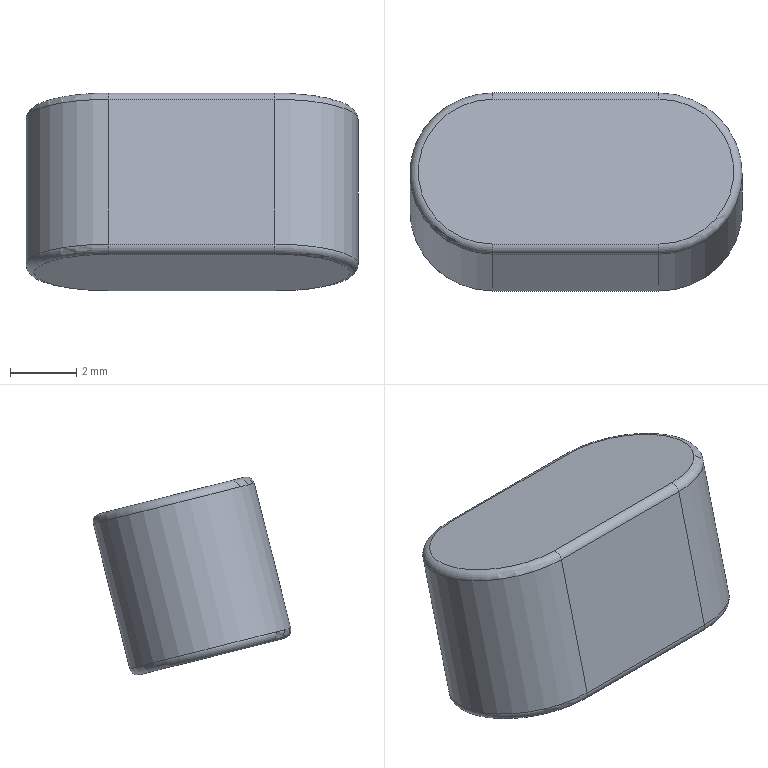Component | NX | STANDARD_FLAT_KEY_A_5X5X10 | 1 solid | 14 faces | box 10 x 5.96 x 5.96 mm | volume 222 mm3 | cylinder 6 | plane 4 | torus 4 | commonest cylinder face diameters 0.5 x4 5 x2
STEP:
#1=CARTESIAN_POINT('',(0.,0.,0.));
#2=DIRECTION('',(0.,0.,1.));
#3=DIRECTION('',(1.,0.,0.));
#4=AXIS2_PLACEMENT_3D('',#1,#2,#3);
#5=CARTESIAN_POINT('',(-1.948,67.926,64.209));
#6=VERTEX_POINT('',#5);
#7=CARTESIAN_POINT('',(-1.948,69.023,68.574));
#8=VERTEX_POINT('',#7);
#9=CARTESIAN_POINT('',(-1.948,67.865,63.967));
#10=DIRECTION('',(0.,0.2438,0.9698));
#11=VECTOR('',#10,1.);
#12=LINE('',#9,#11);
#13=CARTESIAN_POINT('',(-1.948,67.865,63.967));
#14=DIRECTION('',(0.,0.9698,-0.2438));
#15=DIRECTION('',(1.,-0.,0.));
#16=AXIS2_PLACEMENT_3D('',#13,#14,#15);
#17=PLANE('',#16);
#18=CARTESIAN_POINT('',(0.,0.));
#19=DIRECTION('',(-0.,-1.));
#20=VECTOR('',#19,1.);
#21=LINE('',#18,#20);
#22=(GEOMETRIC_REPRESENTATION_CONTEXT(2)PARAMETRIC_REPRESENTATION_CONTEXT()REPRESENTATION_CONTEXT('',''));
#23=DEFINITIONAL_REPRESENTATION('',(#21),#22);
#24=PCURVE('',#17,#23);
#25=CARTESIAN_POINT('',(-1.948,65.44,64.576));
#26=DIRECTION('',(0.,0.2438,0.9698));
#27=DIRECTION('',(-1.,0.,0.));
#28=AXIS2_PLACEMENT_3D('',#25,#26,#27);
#29=CYLINDRICAL_SURFACE('',#28,2.5);
#30=CARTESIAN_POINT('',(4.712,-0.));
#31=DIRECTION('',(0.,1.));
#32=VECTOR('',#31,1.);
#33=LINE('',#30,#32);
#34=(GEOMETRIC_REPRESENTATION_CONTEXT(2)PARAMETRIC_REPRESENTATION_CONTEXT()REPRESENTATION_CONTEXT('',''));
#35=DEFINITIONAL_REPRESENTATION('',(#33),#34);
#36=PCURVE('',#29,#35);
#37=SURFACE_CURVE('',#12,(#24,#36),.PCURVE_S1.);
#38=EDGE_CURVE('',#6,#8,#37,.T.);
#39=ORIENTED_EDGE('',*,*,#38,.F.);
#40=CARTESIAN_POINT('',(-6.948,67.926,64.209));
#41=VERTEX_POINT('',#40);
#42=CARTESIAN_POINT('',(-6.948,67.926,64.209));
#43=DIRECTION('',(-1.,0.,-0.));
#44=VECTOR('',#43,1.);
#45=LINE('',#42,#44);
#46=CARTESIAN_POINT('',(-5.,-0.25));
#47=DIRECTION('',(-1.,0.));
#48=VECTOR('',#47,1.);
#49=LINE('',#46,#48);
#50=(GEOMETRIC_REPRESENTATION_CONTEXT(2)PARAMETRIC_REPRESENTATION_CONTEXT()REPRESENTATION_CONTEXT('',''));
#51=DEFINITIONAL_REPRESENTATION('',(#49),#50);
#52=PCURVE('',#17,#51);
#53=CARTESIAN_POINT('',(-1.948,67.683,64.27));
#54=DIRECTION('',(1.,-0.,0.));
#55=DIRECTION('',(-0.,-0.9698,0.2438));
#56=AXIS2_PLACEMENT_3D('',#53,#54,#55);
#57=CYLINDRICAL_SURFACE('',#56,0.25);
#58=CARTESIAN_POINT('',(3.142,-5.));
#59=DIRECTION('',(0.,-1.));
#60=VECTOR('',#59,1.);
#61=LINE('',#58,#60);
#62=(GEOMETRIC_REPRESENTATION_CONTEXT(2)PARAMETRIC_REPRESENTATION_CONTEXT()REPRESENTATION_CONTEXT('',''));
#63=DEFINITIONAL_REPRESENTATION('',(#61),#62);
#64=PCURVE('',#57,#63);
#65=SURFACE_CURVE('',#45,(#52,#64),.PCURVE_S1.);
#66=EDGE_CURVE('',#6,#41,#65,.T.);
#67=ORIENTED_EDGE('',*,*,#66,.T.);
#68=CARTESIAN_POINT('',(-6.948,69.023,68.574));
#69=VERTEX_POINT('',#68);
#70=CARTESIAN_POINT('',(-6.948,67.865,63.967));
#71=DIRECTION('',(0.,0.2438,0.9698));
#72=VECTOR('',#71,1.);
#73=LINE('',#70,#72);
#74=CARTESIAN_POINT('',(-5.,0.));
#75=DIRECTION('',(-0.,-1.));
#76=VECTOR('',#75,1.);
#77=LINE('',#74,#76);
#78=(GEOMETRIC_REPRESENTATION_CONTEXT(2)PARAMETRIC_REPRESENTATION_CONTEXT()REPRESENTATION_CONTEXT('',''));
#79=DEFINITIONAL_REPRESENTATION('',(#77),#78);
#80=PCURVE('',#17,#79);
#81=CARTESIAN_POINT('',(-6.948,65.44,64.576));
#82=DIRECTION('',(0.,0.2438,0.9698));
#83=DIRECTION('',(-1.,0.,0.));
#84=AXIS2_PLACEMENT_3D('',#81,#82,#83);
#85=CYLINDRICAL_SURFACE('',#84,2.5);
#86=CARTESIAN_POINT('',(-1.571,-0.));
#87=DIRECTION('',(0.,1.));
#88=VECTOR('',#87,1.);
#89=LINE('',#86,#88);
#90=(GEOMETRIC_REPRESENTATION_CONTEXT(2)PARAMETRIC_REPRESENTATION_CONTEXT()REPRESENTATION_CONTEXT('',''));
#91=DEFINITIONAL_REPRESENTATION('',(#89),#90);
#92=PCURVE('',#85,#91);
#93=SURFACE_CURVE('',#73,(#80,#92),.PCURVE_S1.);
#94=EDGE_CURVE('',#41,#69,#93,.T.);
#95=ORIENTED_EDGE('',*,*,#94,.T.);
#96=CARTESIAN_POINT('',(-1.948,69.023,68.574));
#97=DIRECTION('',(1.,-0.,0.));
#98=VECTOR('',#97,1.);
#99=LINE('',#96,#98);
#100=CARTESIAN_POINT('',(-0.,-4.75));
#101=DIRECTION('',(1.,-0.));
#102=VECTOR('',#101,1.);
#103=LINE('',#100,#102);
#104=(GEOMETRIC_REPRESENTATION_CONTEXT(2)PARAMETRIC_REPRESENTATION_CONTEXT()REPRESENTATION_CONTEXT('',''));
#105=DEFINITIONAL_REPRESENTATION('',(#103),#104);
#106=PCURVE('',#17,#105);
#107=CARTESIAN_POINT('',(-6.948,68.78,68.635));
#108=DIRECTION('',(-1.,0.,-0.));
#109=DIRECTION('',(0.,0.9698,-0.2438));
#110=AXIS2_PLACEMENT_3D('',#107,#108,#109);
#111=CYLINDRICAL_SURFACE('',#110,0.25);
#112=CARTESIAN_POINT('',(6.283,-5.));
#113=DIRECTION('',(0.,-1.));
#114=VECTOR('',#113,1.);
#115=LINE('',#112,#114);
#116=(GEOMETRIC_REPRESENTATION_CONTEXT(2)PARAMETRIC_REPRESENTATION_CONTEXT()REPRESENTATION_CONTEXT('',''));
#117=DEFINITIONAL_REPRESENTATION('',(#115),#116);
#118=PCURVE('',#111,#117);
#119=SURFACE_CURVE('',#99,(#106,#118),.PCURVE_S1.);
#120=EDGE_CURVE('',#69,#8,#119,.T.);
#121=ORIENTED_EDGE('',*,*,#120,.T.);
#122=EDGE_LOOP('',(#39,#67,#95,#121));
#123=FACE_BOUND('',#122,.T.);
#124=ADVANCED_FACE('',(#123),#17,.T.);
#125=ORIENTED_EDGE('',*,*,#94,.F.);
#126=CARTESIAN_POINT('',(-6.948,63.077,65.428));
#127=VERTEX_POINT('',#126);
#128=CARTESIAN_POINT('',(-6.948,65.501,64.819));
#129=DIRECTION('',(0.,0.2438,0.9698));
#130=DIRECTION('',(-1.,0.,0.));
#131=AXIS2_PLACEMENT_3D('',#128,#129,#130);
#132=CIRCLE('',#131,2.5);
#133=CARTESIAN_POINT('',(-6.283,0.25));
#134=DIRECTION('',(1.,0.));
#135=VECTOR('',#134,1.);
#136=LINE('',#133,#135);
#137=(GEOMETRIC_REPRESENTATION_CONTEXT(2)PARAMETRIC_REPRESENTATION_CONTEXT()REPRESENTATION_CONTEXT('',''));
#138=DEFINITIONAL_REPRESENTATION('',(#136),#137);
#139=PCURVE('',#85,#138);
#140=CARTESIAN_POINT('',(-6.948,65.501,64.819));
#141=DIRECTION('',(0.,0.2438,0.9698));
#142=DIRECTION('',(-1.,0.,0.));
#143=AXIS2_PLACEMENT_3D('',#140,#141,#142);
#144=TOROIDAL_SURFACE('',#143,2.25,0.25);
#145=CARTESIAN_POINT('',(-6.283,6.283));
#146=DIRECTION('',(1.,0.));
#147=VECTOR('',#146,1.);
#148=LINE('',#145,#147);
#149=(GEOMETRIC_REPRESENTATION_CONTEXT(2)PARAMETRIC_REPRESENTATION_CONTEXT()REPRESENTATION_CONTEXT('',''));
#150=DEFINITIONAL_REPRESENTATION('',(#148),#149);
#151=PCURVE('',#144,#150);
#152=SURFACE_CURVE('',#132,(#139,#151),.PCURVE_S1.);
#153=EDGE_CURVE('',#41,#127,#152,.T.);
#154=ORIENTED_EDGE('',*,*,#153,.T.);
#155=CARTESIAN_POINT('',(-6.948,64.174,69.793));
#156=VERTEX_POINT('',#155);
#157=CARTESIAN_POINT('',(-6.948,63.016,65.186));
#158=DIRECTION('',(0.,0.2438,0.9698));
#159=VECTOR('',#158,1.);
#160=LINE('',#157,#159);
#161=CARTESIAN_POINT('',(1.571,0.));
#162=DIRECTION('',(0.,1.));
#163=VECTOR('',#162,1.);
#164=LINE('',#161,#163);
#165=(GEOMETRIC_REPRESENTATION_CONTEXT(2)PARAMETRIC_REPRESENTATION_CONTEXT()REPRESENTATION_CONTEXT('',''));
#166=DEFINITIONAL_REPRESENTATION('',(#164),#165);
#167=PCURVE('',#85,#166);
#168=CARTESIAN_POINT('',(-6.948,63.016,65.186));
#169=DIRECTION('',(0.,-0.9698,0.2438));
#170=DIRECTION('',(0.,-0.2438,-0.9698));
#171=AXIS2_PLACEMENT_3D('',#168,#169,#170);
#172=PLANE('',#171);
#173=CARTESIAN_POINT('',(-0.,0.));
#174=DIRECTION('',(-1.,0.));
#175=VECTOR('',#174,1.);
#176=LINE('',#173,#175);
#177=(GEOMETRIC_REPRESENTATION_CONTEXT(2)PARAMETRIC_REPRESENTATION_CONTEXT()REPRESENTATION_CONTEXT('',''));
#178=DEFINITIONAL_REPRESENTATION('',(#176),#177);
#179=PCURVE('',#172,#178);
#180=SURFACE_CURVE('',#160,(#167,#179),.PCURVE_S1.);
#181=EDGE_CURVE('',#127,#156,#180,.T.);
#182=ORIENTED_EDGE('',*,*,#181,.T.);
#183=CARTESIAN_POINT('',(-6.948,66.598,69.183));
#184=DIRECTION('',(0.,-0.2438,-0.9698));
#185=DIRECTION('',(-1.,0.,0.));
#186=AXIS2_PLACEMENT_3D('',#183,#184,#185);
#187=CIRCLE('',#186,2.5);
#188=CARTESIAN_POINT('',(6.283,4.75));
#189=DIRECTION('',(-1.,0.));
#190=VECTOR('',#189,1.);
#191=LINE('',#188,#190);
#192=(GEOMETRIC_REPRESENTATION_CONTEXT(2)PARAMETRIC_REPRESENTATION_CONTEXT()REPRESENTATION_CONTEXT('',''));
#193=DEFINITIONAL_REPRESENTATION('',(#191),#192);
#194=PCURVE('',#85,#193);
#195=CARTESIAN_POINT('',(-6.948,66.598,69.183));
#196=DIRECTION('',(0.,0.2438,0.9698));
#197=DIRECTION('',(-1.,0.,0.));
#198=AXIS2_PLACEMENT_3D('',#195,#196,#197);
#199=TOROIDAL_SURFACE('',#198,2.25,0.25);
#200=CARTESIAN_POINT('',(6.283,0.));
#201=DIRECTION('',(-1.,0.));
#202=VECTOR('',#201,1.);
#203=LINE('',#200,#202);
#204=(GEOMETRIC_REPRESENTATION_CONTEXT(2)PARAMETRIC_REPRESENTATION_CONTEXT()REPRESENTATION_CONTEXT('',''));
#205=DEFINITIONAL_REPRESENTATION('',(#203),#204);
#206=PCURVE('',#199,#205);
#207=SURFACE_CURVE('',#187,(#194,#206),.PCURVE_S1.);
#208=EDGE_CURVE('',#156,#69,#207,.T.);
#209=ORIENTED_EDGE('',*,*,#208,.T.);
#210=EDGE_LOOP('',(#125,#154,#182,#209));
#211=FACE_BOUND('',#210,.T.);
#212=ADVANCED_FACE('',(#211),#85,.T.);
#213=ORIENTED_EDGE('',*,*,#181,.F.);
#214=CARTESIAN_POINT('',(-1.948,63.077,65.428));
#215=VERTEX_POINT('',#214);
#216=CARTESIAN_POINT('',(-1.948,63.077,65.428));
#217=DIRECTION('',(1.,0.,0.));
#218=VECTOR('',#217,1.);
#219=LINE('',#216,#218);
#220=CARTESIAN_POINT('',(-0.25,5.));
#221=DIRECTION('',(0.,1.));
#222=VECTOR('',#221,1.);
#223=LINE('',#220,#222);
#224=(GEOMETRIC_REPRESENTATION_CONTEXT(2)PARAMETRIC_REPRESENTATION_CONTEXT()REPRESENTATION_CONTEXT('',''));
#225=DEFINITIONAL_REPRESENTATION('',(#223),#224);
#226=PCURVE('',#172,#225);
#227=CARTESIAN_POINT('',(-6.948,63.319,65.367));
#228=DIRECTION('',(-1.,0.,0.));
#229=DIRECTION('',(0.,-0.2438,-0.9698));
#230=AXIS2_PLACEMENT_3D('',#227,#228,#229);
#231=CYLINDRICAL_SURFACE('',#230,0.25);
#232=CARTESIAN_POINT('',(1.571,-5.));
#233=DIRECTION('',(0.,-1.));
#234=VECTOR('',#233,1.);
#235=LINE('',#232,#234);
#236=(GEOMETRIC_REPRESENTATION_CONTEXT(2)PARAMETRIC_REPRESENTATION_CONTEXT()REPRESENTATION_CONTEXT('',''));
#237=DEFINITIONAL_REPRESENTATION('',(#235),#236);
#238=PCURVE('',#231,#237);
#239=SURFACE_CURVE('',#219,(#226,#238),.PCURVE_S1.);
#240=EDGE_CURVE('',#127,#215,#239,.T.);
#241=ORIENTED_EDGE('',*,*,#240,.T.);
#242=CARTESIAN_POINT('',(-1.948,64.174,69.793));
#243=VERTEX_POINT('',#242);
#244=CARTESIAN_POINT('',(-1.948,63.016,65.186));
#245=DIRECTION('',(0.,0.2438,0.9698));
#246=VECTOR('',#245,1.);
#247=LINE('',#244,#246);
#248=CARTESIAN_POINT('',(0.,5.));
#249=DIRECTION('',(-1.,0.));
#250=VECTOR('',#249,1.);
#251=LINE('',#248,#250);
#252=(GEOMETRIC_REPRESENTATION_CONTEXT(2)PARAMETRIC_REPRESENTATION_CONTEXT()REPRESENTATION_CONTEXT('',''));
#253=DEFINITIONAL_REPRESENTATION('',(#251),#252);
#254=PCURVE('',#172,#253);
#255=CARTESIAN_POINT('',(1.571,0.));
#256=DIRECTION('',(0.,1.));
#257=VECTOR('',#256,1.);
#258=LINE('',#255,#257);
#259=(GEOMETRIC_REPRESENTATION_CONTEXT(2)PARAMETRIC_REPRESENTATION_CONTEXT()REPRESENTATION_CONTEXT('',''));
#260=DEFINITIONAL_REPRESENTATION('',(#258),#259);
#261=PCURVE('',#29,#260);
#262=SURFACE_CURVE('',#247,(#254,#261),.PCURVE_S1.);
#263=EDGE_CURVE('',#215,#243,#262,.T.);
#264=ORIENTED_EDGE('',*,*,#263,.T.);
#265=CARTESIAN_POINT('',(-6.948,64.174,69.793));
#266=DIRECTION('',(-1.,0.,0.));
#267=VECTOR('',#266,1.);
#268=LINE('',#265,#267);
#269=CARTESIAN_POINT('',(-4.75,0.));
#270=DIRECTION('',(0.,-1.));
#271=VECTOR('',#270,1.);
#272=LINE('',#269,#271);
#273=(GEOMETRIC_REPRESENTATION_CONTEXT(2)PARAMETRIC_REPRESENTATION_CONTEXT()REPRESENTATION_CONTEXT('',''));
#274=DEFINITIONAL_REPRESENTATION('',(#272),#273);
#275=PCURVE('',#172,#274);
#276=CARTESIAN_POINT('',(-6.948,64.416,69.732));
#277=DIRECTION('',(1.,0.,0.));
#278=DIRECTION('',(0.,0.2438,0.9698));
#279=AXIS2_PLACEMENT_3D('',#276,#277,#278);
#280=CYLINDRICAL_SURFACE('',#279,0.25);
#281=CARTESIAN_POINT('',(1.571,0.));
#282=DIRECTION('',(0.,-1.));
#283=VECTOR('',#282,1.);
#284=LINE('',#281,#283);
#285=(GEOMETRIC_REPRESENTATION_CONTEXT(2)PARAMETRIC_REPRESENTATION_CONTEXT()REPRESENTATION_CONTEXT('',''));
#286=DEFINITIONAL_REPRESENTATION('',(#284),#285);
#287=PCURVE('',#280,#286);
#288=SURFACE_CURVE('',#268,(#275,#287),.PCURVE_S1.);
#289=EDGE_CURVE('',#243,#156,#288,.T.);
#290=ORIENTED_EDGE('',*,*,#289,.T.);
#291=EDGE_LOOP('',(#213,#241,#264,#290));
#292=FACE_BOUND('',#291,.T.);
#293=ADVANCED_FACE('',(#292),#172,.T.);
#294=ORIENTED_EDGE('',*,*,#263,.F.);
#295=CARTESIAN_POINT('',(-1.948,65.501,64.819));
#296=DIRECTION('',(0.,0.2438,0.9698));
#297=DIRECTION('',(-1.,0.,0.));
#298=AXIS2_PLACEMENT_3D('',#295,#296,#297);
#299=CIRCLE('',#298,2.5);
#300=CARTESIAN_POINT('',(0.,0.25));
#301=DIRECTION('',(1.,0.));
#302=VECTOR('',#301,1.);
#303=LINE('',#300,#302);
#304=(GEOMETRIC_REPRESENTATION_CONTEXT(2)PARAMETRIC_REPRESENTATION_CONTEXT()REPRESENTATION_CONTEXT('',''));
#305=DEFINITIONAL_REPRESENTATION('',(#303),#304);
#306=PCURVE('',#29,#305);
#307=CARTESIAN_POINT('',(-1.948,65.501,64.819));
#308=DIRECTION('',(0.,0.2438,0.9698));
#309=DIRECTION('',(-1.,0.,0.));
#310=AXIS2_PLACEMENT_3D('',#307,#308,#309);
#311=TOROIDAL_SURFACE('',#310,2.25,0.25);
#312=CARTESIAN_POINT('',(0.,6.283));
#313=DIRECTION('',(1.,0.));
#314=VECTOR('',#313,1.);
#315=LINE('',#312,#314);
#316=(GEOMETRIC_REPRESENTATION_CONTEXT(2)PARAMETRIC_REPRESENTATION_CONTEXT()REPRESENTATION_CONTEXT('',''));
#317=DEFINITIONAL_REPRESENTATION('',(#315),#316);
#318=PCURVE('',#311,#317);
#319=SURFACE_CURVE('',#299,(#306,#318),.PCURVE_S1.);
#320=EDGE_CURVE('',#215,#6,#319,.T.);
#321=ORIENTED_EDGE('',*,*,#320,.T.);
#322=ORIENTED_EDGE('',*,*,#38,.T.);
#323=CARTESIAN_POINT('',(-1.948,66.598,69.183));
#324=DIRECTION('',(0.,-0.2438,-0.9698));
#325=DIRECTION('',(-1.,0.,0.));
#326=AXIS2_PLACEMENT_3D('',#323,#324,#325);
#327=CIRCLE('',#326,2.5);
#328=CARTESIAN_POINT('',(6.283,4.75));
#329=DIRECTION('',(-1.,0.));
#330=VECTOR('',#329,1.);
#331=LINE('',#328,#330);
#332=(GEOMETRIC_REPRESENTATION_CONTEXT(2)PARAMETRIC_REPRESENTATION_CONTEXT()REPRESENTATION_CONTEXT('',''));
#333=DEFINITIONAL_REPRESENTATION('',(#331),#332);
#334=PCURVE('',#29,#333);
#335=CARTESIAN_POINT('',(-1.948,66.598,69.183));
#336=DIRECTION('',(0.,0.2438,0.9698));
#337=DIRECTION('',(-1.,0.,0.));
#338=AXIS2_PLACEMENT_3D('',#335,#336,#337);
#339=TOROIDAL_SURFACE('',#338,2.25,0.25);
#340=CARTESIAN_POINT('',(6.283,0.));
#341=DIRECTION('',(-1.,0.));
#342=VECTOR('',#341,1.);
#343=LINE('',#340,#342);
#344=(GEOMETRIC_REPRESENTATION_CONTEXT(2)PARAMETRIC_REPRESENTATION_CONTEXT()REPRESENTATION_CONTEXT('',''));
#345=DEFINITIONAL_REPRESENTATION('',(#343),#344);
#346=PCURVE('',#339,#345);
#347=SURFACE_CURVE('',#327,(#334,#346),.PCURVE_S1.);
#348=EDGE_CURVE('',#8,#243,#347,.T.);
#349=ORIENTED_EDGE('',*,*,#348,.T.);
#350=EDGE_LOOP('',(#294,#321,#322,#349));
#351=FACE_BOUND('',#350,.T.);
#352=ADVANCED_FACE('',(#351),#29,.T.);
#353=CARTESIAN_POINT('',(-1.948,67.622,64.028));
#354=VERTEX_POINT('',#353);
#355=CARTESIAN_POINT('',(-1.948,63.258,65.125));
#356=VERTEX_POINT('',#355);
#357=CARTESIAN_POINT('',(-1.948,65.44,64.576));
#358=DIRECTION('',(0.,-0.2438,-0.9698));
#359=DIRECTION('',(-1.,0.,0.));
#360=AXIS2_PLACEMENT_3D('',#357,#358,#359);
#361=CIRCLE('',#360,2.25);
#362=CARTESIAN_POINT('',(-6.948,65.44,64.576));
#363=DIRECTION('',(0.,0.2438,0.9698));
#364=DIRECTION('',(-1.,0.,0.));
#365=AXIS2_PLACEMENT_3D('',#362,#363,#364);
#366=PLANE('',#365);
#367=CARTESIAN_POINT('',(-2.75,0.));
#368=CARTESIAN_POINT('',(-2.75,-3.897));
#369=CARTESIAN_POINT('',(-6.125,-1.949));
#370=CARTESIAN_POINT('',(-9.5,-0.));
#371=CARTESIAN_POINT('',(-6.125,1.949));
#372=CARTESIAN_POINT('',(-2.75,3.897));
#373=CARTESIAN_POINT('',(-2.75,0.));
#374=(BOUNDED_CURVE()B_SPLINE_CURVE(2,(#367,#368,#369,#370,#371,#372,#373),.UNSPECIFIED.,.T.,.F.)B_SPLINE_CURVE_WITH_KNOTS((1,2,2,2,2,1),(-2.094,0.,2.094,4.189,6.283,8.378),.UNSPECIFIED.)CURVE()GEOMETRIC_REPRESENTATION_ITEM()RATIONAL_B_SPLINE_CURVE((1.,0.5,1.,0.5,1.,0.5,1.))REPRESENTATION_ITEM(''));
#375=(GEOMETRIC_REPRESENTATION_CONTEXT(2)PARAMETRIC_REPRESENTATION_CONTEXT()REPRESENTATION_CONTEXT('',''));
#376=DEFINITIONAL_REPRESENTATION('',(#374),#375);
#377=PCURVE('',#366,#376);
#378=CARTESIAN_POINT('',(6.283,4.712));
#379=DIRECTION('',(-1.,-0.));
#380=VECTOR('',#379,1.);
#381=LINE('',#378,#380);
#382=(GEOMETRIC_REPRESENTATION_CONTEXT(2)PARAMETRIC_REPRESENTATION_CONTEXT()REPRESENTATION_CONTEXT('',''));
#383=DEFINITIONAL_REPRESENTATION('',(#381),#382);
#384=PCURVE('',#311,#383);
#385=SURFACE_CURVE('',#361,(#377,#384),.PCURVE_S1.);
#386=EDGE_CURVE('',#354,#356,#385,.T.);
#387=ORIENTED_EDGE('',*,*,#386,.T.);
#388=CARTESIAN_POINT('',(-6.948,63.258,65.125));
#389=VERTEX_POINT('',#388);
#390=CARTESIAN_POINT('',(-6.948,63.258,65.125));
#391=DIRECTION('',(-1.,0.,0.));
#392=VECTOR('',#391,1.);
#393=LINE('',#390,#392);
#394=CARTESIAN_POINT('',(0.,2.25));
#395=DIRECTION('',(1.,0.));
#396=VECTOR('',#395,1.);
#397=LINE('',#394,#396);
#398=(GEOMETRIC_REPRESENTATION_CONTEXT(2)PARAMETRIC_REPRESENTATION_CONTEXT()REPRESENTATION_CONTEXT('',''));
#399=DEFINITIONAL_REPRESENTATION('',(#397),#398);
#400=PCURVE('',#366,#399);
#401=CARTESIAN_POINT('',(0.,0.));
#402=DIRECTION('',(0.,1.));
#403=VECTOR('',#402,1.);
#404=LINE('',#401,#403);
#405=(GEOMETRIC_REPRESENTATION_CONTEXT(2)PARAMETRIC_REPRESENTATION_CONTEXT()REPRESENTATION_CONTEXT('',''));
#406=DEFINITIONAL_REPRESENTATION('',(#404),#405);
#407=PCURVE('',#231,#406);
#408=SURFACE_CURVE('',#393,(#400,#407),.PCURVE_S1.);
#409=EDGE_CURVE('',#356,#389,#408,.T.);
#410=ORIENTED_EDGE('',*,*,#409,.T.);
#411=CARTESIAN_POINT('',(-6.948,67.622,64.028));
#412=VERTEX_POINT('',#411);
#413=CARTESIAN_POINT('',(-6.948,65.44,64.576));
#414=DIRECTION('',(0.,-0.2438,-0.9698));
#415=DIRECTION('',(-1.,0.,0.));
#416=AXIS2_PLACEMENT_3D('',#413,#414,#415);
#417=CIRCLE('',#416,2.25);
#418=CARTESIAN_POINT('',(2.25,0.));
#419=CARTESIAN_POINT('',(2.25,-3.897));
#420=CARTESIAN_POINT('',(-1.125,-1.949));
#421=CARTESIAN_POINT('',(-4.5,-0.));
#422=CARTESIAN_POINT('',(-1.125,1.949));
#423=CARTESIAN_POINT('',(2.25,3.897));
#424=CARTESIAN_POINT('',(2.25,0.));
#425=(BOUNDED_CURVE()B_SPLINE_CURVE(2,(#418,#419,#420,#421,#422,#423,#424),.UNSPECIFIED.,.T.,.F.)B_SPLINE_CURVE_WITH_KNOTS((1,2,2,2,2,1),(-2.094,0.,2.094,4.189,6.283,8.378),.UNSPECIFIED.)CURVE()GEOMETRIC_REPRESENTATION_ITEM()RATIONAL_B_SPLINE_CURVE((1.,0.5,1.,0.5,1.,0.5,1.))REPRESENTATION_ITEM(''));
#426=(GEOMETRIC_REPRESENTATION_CONTEXT(2)PARAMETRIC_REPRESENTATION_CONTEXT()REPRESENTATION_CONTEXT('',''));
#427=DEFINITIONAL_REPRESENTATION('',(#425),#426);
#428=PCURVE('',#366,#427);
#429=CARTESIAN_POINT('',(6.283,4.712));
#430=DIRECTION('',(-1.,0.));
#431=VECTOR('',#430,1.);
#432=LINE('',#429,#431);
#433=(GEOMETRIC_REPRESENTATION_CONTEXT(2)PARAMETRIC_REPRESENTATION_CONTEXT()REPRESENTATION_CONTEXT('',''));
#434=DEFINITIONAL_REPRESENTATION('',(#432),#433);
#435=PCURVE('',#144,#434);
#436=SURFACE_CURVE('',#417,(#428,#435),.PCURVE_S1.);
#437=EDGE_CURVE('',#389,#412,#436,.T.);
#438=ORIENTED_EDGE('',*,*,#437,.T.);
#439=CARTESIAN_POINT('',(-1.948,67.622,64.028));
#440=DIRECTION('',(1.,-0.,0.));
#441=VECTOR('',#440,1.);
#442=LINE('',#439,#441);
#443=CARTESIAN_POINT('',(-5.,-2.25));
#444=DIRECTION('',(-1.,0.));
#445=VECTOR('',#444,1.);
#446=LINE('',#443,#445);
#447=(GEOMETRIC_REPRESENTATION_CONTEXT(2)PARAMETRIC_REPRESENTATION_CONTEXT()REPRESENTATION_CONTEXT('',''));
#448=DEFINITIONAL_REPRESENTATION('',(#446),#447);
#449=PCURVE('',#366,#448);
#450=CARTESIAN_POINT('',(1.571,0.));
#451=DIRECTION('',(0.,1.));
#452=VECTOR('',#451,1.);
#453=LINE('',#450,#452);
#454=(GEOMETRIC_REPRESENTATION_CONTEXT(2)PARAMETRIC_REPRESENTATION_CONTEXT()REPRESENTATION_CONTEXT('',''));
#455=DEFINITIONAL_REPRESENTATION('',(#453),#454);
#456=PCURVE('',#57,#455);
#457=SURFACE_CURVE('',#442,(#449,#456),.PCURVE_S1.);
#458=EDGE_CURVE('',#412,#354,#457,.T.);
#459=ORIENTED_EDGE('',*,*,#458,.T.);
#460=EDGE_LOOP('',(#387,#410,#438,#459));
#461=FACE_BOUND('',#460,.T.);
#462=ADVANCED_FACE('',(#461),#366,.F.);
#463=CARTESIAN_POINT('',(-6.948,68.841,68.877));
#464=VERTEX_POINT('',#463);
#465=CARTESIAN_POINT('',(-6.948,64.477,69.974));
#466=VERTEX_POINT('',#465);
#467=CARTESIAN_POINT('',(-6.948,66.659,69.426));
#468=DIRECTION('',(0.,0.2438,0.9698));
#469=DIRECTION('',(-1.,0.,0.));
#470=AXIS2_PLACEMENT_3D('',#467,#468,#469);
#471=CIRCLE('',#470,2.25);
#472=CARTESIAN_POINT('',(-6.948,66.659,69.426));
#473=DIRECTION('',(0.,0.2438,0.9698));
#474=DIRECTION('',(-1.,0.,0.));
#475=AXIS2_PLACEMENT_3D('',#472,#473,#474);
#476=PLANE('',#475);
#477=CARTESIAN_POINT('',(0.,0.));
#478=DIRECTION('',(1.,0.));
#479=AXIS2_PLACEMENT_2D('',#477,#478);
#480=CIRCLE('',#479,2.25);
#481=(GEOMETRIC_REPRESENTATION_CONTEXT(2)PARAMETRIC_REPRESENTATION_CONTEXT()REPRESENTATION_CONTEXT('',''));
#482=DEFINITIONAL_REPRESENTATION('',(#480),#481);
#483=PCURVE('',#476,#482);
#484=CARTESIAN_POINT('',(-6.283,1.571));
#485=DIRECTION('',(1.,-0.));
#486=VECTOR('',#485,1.);
#487=LINE('',#484,#486);
#488=(GEOMETRIC_REPRESENTATION_CONTEXT(2)PARAMETRIC_REPRESENTATION_CONTEXT()REPRESENTATION_CONTEXT('',''));
#489=DEFINITIONAL_REPRESENTATION('',(#487),#488);
#490=PCURVE('',#199,#489);
#491=SURFACE_CURVE('',#471,(#483,#490),.PCURVE_S1.);
#492=EDGE_CURVE('',#464,#466,#491,.T.);
#493=ORIENTED_EDGE('',*,*,#492,.T.);
#494=CARTESIAN_POINT('',(-1.948,64.477,69.974));
#495=VERTEX_POINT('',#494);
#496=CARTESIAN_POINT('',(-6.948,64.477,69.974));
#497=DIRECTION('',(1.,0.,0.));
#498=VECTOR('',#497,1.);
#499=LINE('',#496,#498);
#500=CARTESIAN_POINT('',(0.,2.25));
#501=DIRECTION('',(-1.,0.));
#502=VECTOR('',#501,1.);
#503=LINE('',#500,#502);
#504=(GEOMETRIC_REPRESENTATION_CONTEXT(2)PARAMETRIC_REPRESENTATION_CONTEXT()REPRESENTATION_CONTEXT('',''));
#505=DEFINITIONAL_REPRESENTATION('',(#503),#504);
#506=PCURVE('',#476,#505);
#507=CARTESIAN_POINT('',(0.,0.));
#508=DIRECTION('',(0.,1.));
#509=VECTOR('',#508,1.);
#510=LINE('',#507,#509);
#511=(GEOMETRIC_REPRESENTATION_CONTEXT(2)PARAMETRIC_REPRESENTATION_CONTEXT()REPRESENTATION_CONTEXT('',''));
#512=DEFINITIONAL_REPRESENTATION('',(#510),#511);
#513=PCURVE('',#280,#512);
#514=SURFACE_CURVE('',#499,(#506,#513),.PCURVE_S1.);
#515=EDGE_CURVE('',#466,#495,#514,.T.);
#516=ORIENTED_EDGE('',*,*,#515,.T.);
#517=CARTESIAN_POINT('',(-1.948,68.841,68.877));
#518=VERTEX_POINT('',#517);
#519=CARTESIAN_POINT('',(-1.948,66.659,69.426));
#520=DIRECTION('',(0.,0.2438,0.9698));
#521=DIRECTION('',(-1.,0.,0.));
#522=AXIS2_PLACEMENT_3D('',#519,#520,#521);
#523=CIRCLE('',#522,2.25);
#524=CARTESIAN_POINT('',(-5.,0.));
#525=DIRECTION('',(1.,0.));
#526=AXIS2_PLACEMENT_2D('',#524,#525);
#527=CIRCLE('',#526,2.25);
#528=(GEOMETRIC_REPRESENTATION_CONTEXT(2)PARAMETRIC_REPRESENTATION_CONTEXT()REPRESENTATION_CONTEXT('',''));
#529=DEFINITIONAL_REPRESENTATION('',(#527),#528);
#530=PCURVE('',#476,#529);
#531=CARTESIAN_POINT('',(0.,1.571));
#532=DIRECTION('',(1.,0.));
#533=VECTOR('',#532,1.);
#534=LINE('',#531,#533);
#535=(GEOMETRIC_REPRESENTATION_CONTEXT(2)PARAMETRIC_REPRESENTATION_CONTEXT()REPRESENTATION_CONTEXT('',''));
#536=DEFINITIONAL_REPRESENTATION('',(#534),#535);
#537=PCURVE('',#339,#536);
#538=SURFACE_CURVE('',#523,(#530,#537),.PCURVE_S1.);
#539=EDGE_CURVE('',#495,#518,#538,.T.);
#540=ORIENTED_EDGE('',*,*,#539,.T.);
#541=CARTESIAN_POINT('',(-6.948,68.841,68.877));
#542=DIRECTION('',(-1.,0.,-0.));
#543=VECTOR('',#542,1.);
#544=LINE('',#541,#543);
#545=CARTESIAN_POINT('',(0.,-2.25));
#546=DIRECTION('',(1.,-0.));
#547=VECTOR('',#546,1.);
#548=LINE('',#545,#547);
#549=(GEOMETRIC_REPRESENTATION_CONTEXT(2)PARAMETRIC_REPRESENTATION_CONTEXT()REPRESENTATION_CONTEXT('',''));
#550=DEFINITIONAL_REPRESENTATION('',(#548),#549);
#551=PCURVE('',#476,#550);
#552=CARTESIAN_POINT('',(4.712,0.));
#553=DIRECTION('',(-0.,1.));
#554=VECTOR('',#553,1.);
#555=LINE('',#552,#554);
#556=(GEOMETRIC_REPRESENTATION_CONTEXT(2)PARAMETRIC_REPRESENTATION_CONTEXT()REPRESENTATION_CONTEXT('',''));
#557=DEFINITIONAL_REPRESENTATION('',(#555),#556);
#558=PCURVE('',#111,#557);
#559=SURFACE_CURVE('',#544,(#551,#558),.PCURVE_S1.);
#560=EDGE_CURVE('',#518,#464,#559,.T.);
#561=ORIENTED_EDGE('',*,*,#560,.T.);
#562=EDGE_LOOP('',(#493,#516,#540,#561));
#563=FACE_BOUND('',#562,.T.);
#564=ADVANCED_FACE('',(#563),#476,.T.);
#565=CARTESIAN_POINT('',(-1.948,67.683,64.27));
#566=DIRECTION('',(1.,-0.,0.));
#567=DIRECTION('',(-0.,-0.9698,0.2438));
#568=AXIS2_PLACEMENT_3D('',#565,#566,#567);
#569=CIRCLE('',#568,0.25);
#570=CARTESIAN_POINT('',(0.,0.));
#571=DIRECTION('',(1.,0.));
#572=VECTOR('',#571,1.);
#573=LINE('',#570,#572);
#574=(GEOMETRIC_REPRESENTATION_CONTEXT(2)PARAMETRIC_REPRESENTATION_CONTEXT()REPRESENTATION_CONTEXT('',''));
#575=DEFINITIONAL_REPRESENTATION('',(#573),#574);
#576=PCURVE('',#57,#575);
#577=CARTESIAN_POINT('',(4.712,3.142));
#578=DIRECTION('',(0.,1.));
#579=VECTOR('',#578,1.);
#580=LINE('',#577,#579);
#581=(GEOMETRIC_REPRESENTATION_CONTEXT(2)PARAMETRIC_REPRESENTATION_CONTEXT()REPRESENTATION_CONTEXT('',''));
#582=DEFINITIONAL_REPRESENTATION('',(#580),#581);
#583=PCURVE('',#311,#582);
#584=SURFACE_CURVE('',#569,(#576,#583),.PCURVE_S1.);
#585=EDGE_CURVE('',#354,#6,#584,.T.);
#586=ORIENTED_EDGE('',*,*,#585,.F.);
#587=ORIENTED_EDGE('',*,*,#458,.F.);
#588=CARTESIAN_POINT('',(-6.948,67.683,64.27));
#589=DIRECTION('',(-1.,0.,-0.));
#590=DIRECTION('',(0.,-0.2438,-0.9698));
#591=AXIS2_PLACEMENT_3D('',#588,#589,#590);
#592=CIRCLE('',#591,0.25);
#593=CARTESIAN_POINT('',(7.854,-5.));
#594=DIRECTION('',(-1.,0.));
#595=VECTOR('',#594,1.);
#596=LINE('',#593,#595);
#597=(GEOMETRIC_REPRESENTATION_CONTEXT(2)PARAMETRIC_REPRESENTATION_CONTEXT()REPRESENTATION_CONTEXT('',''));
#598=DEFINITIONAL_REPRESENTATION('',(#596),#597);
#599=PCURVE('',#57,#598);
#600=CARTESIAN_POINT('',(-1.571,10.996));
#601=DIRECTION('',(0.,-1.));
#602=VECTOR('',#601,1.);
#603=LINE('',#600,#602);
#604=(GEOMETRIC_REPRESENTATION_CONTEXT(2)PARAMETRIC_REPRESENTATION_CONTEXT()REPRESENTATION_CONTEXT('',''));
#605=DEFINITIONAL_REPRESENTATION('',(#603),#604);
#606=PCURVE('',#144,#605);
#607=SURFACE_CURVE('',#592,(#599,#606),.PCURVE_S1.);
#608=EDGE_CURVE('',#41,#412,#607,.T.);
#609=ORIENTED_EDGE('',*,*,#608,.F.);
#610=ORIENTED_EDGE('',*,*,#66,.F.);
#611=EDGE_LOOP('',(#586,#587,#609,#610));
#612=FACE_BOUND('',#611,.T.);
#613=ADVANCED_FACE('',(#612),#57,.T.);
#614=ORIENTED_EDGE('',*,*,#608,.T.);
#615=ORIENTED_EDGE('',*,*,#437,.F.);
#616=CARTESIAN_POINT('',(-6.948,63.319,65.367));
#617=DIRECTION('',(1.,0.,0.));
#618=DIRECTION('',(0.,0.2438,0.9698));
#619=AXIS2_PLACEMENT_3D('',#616,#617,#618);
#620=CIRCLE('',#619,0.25);
#621=CARTESIAN_POINT('',(1.571,7.854));
#622=DIRECTION('',(0.,-1.));
#623=VECTOR('',#622,1.);
#624=LINE('',#621,#623);
#625=(GEOMETRIC_REPRESENTATION_CONTEXT(2)PARAMETRIC_REPRESENTATION_CONTEXT()REPRESENTATION_CONTEXT('',''));
#626=DEFINITIONAL_REPRESENTATION('',(#624),#625);
#627=PCURVE('',#144,#626);
#628=CARTESIAN_POINT('',(3.142,0.));
#629=DIRECTION('',(-1.,0.));
#630=VECTOR('',#629,1.);
#631=LINE('',#628,#630);
#632=(GEOMETRIC_REPRESENTATION_CONTEXT(2)PARAMETRIC_REPRESENTATION_CONTEXT()REPRESENTATION_CONTEXT('',''));
#633=DEFINITIONAL_REPRESENTATION('',(#631),#632);
#634=PCURVE('',#231,#633);
#635=SURFACE_CURVE('',#620,(#627,#634),.PCURVE_S1.);
#636=EDGE_CURVE('',#127,#389,#635,.T.);
#637=ORIENTED_EDGE('',*,*,#636,.F.);
#638=ORIENTED_EDGE('',*,*,#153,.F.);
#639=EDGE_LOOP('',(#614,#615,#637,#638));
#640=FACE_BOUND('',#639,.T.);
#641=ADVANCED_FACE('',(#640),#144,.T.);
#642=ORIENTED_EDGE('',*,*,#585,.T.);
#643=ORIENTED_EDGE('',*,*,#320,.F.);
#644=CARTESIAN_POINT('',(-1.948,63.319,65.367));
#645=DIRECTION('',(-1.,0.,0.));
#646=DIRECTION('',(0.,-0.2438,-0.9698));
#647=AXIS2_PLACEMENT_3D('',#644,#645,#646);
#648=CIRCLE('',#647,0.25);
#649=CARTESIAN_POINT('',(1.571,4.712));
#650=DIRECTION('',(0.,1.));
#651=VECTOR('',#650,1.);
#652=LINE('',#649,#651);
#653=(GEOMETRIC_REPRESENTATION_CONTEXT(2)PARAMETRIC_REPRESENTATION_CONTEXT()REPRESENTATION_CONTEXT('',''));
#654=DEFINITIONAL_REPRESENTATION('',(#652),#653);
#655=PCURVE('',#311,#654);
#656=CARTESIAN_POINT('',(0.,-5.));
#657=DIRECTION('',(1.,0.));
#658=VECTOR('',#657,1.);
#659=LINE('',#656,#658);
#660=(GEOMETRIC_REPRESENTATION_CONTEXT(2)PARAMETRIC_REPRESENTATION_CONTEXT()REPRESENTATION_CONTEXT('',''));
#661=DEFINITIONAL_REPRESENTATION('',(#659),#660);
#662=PCURVE('',#231,#661);
#663=SURFACE_CURVE('',#648,(#655,#662),.PCURVE_S1.);
#664=EDGE_CURVE('',#356,#215,#663,.T.);
#665=ORIENTED_EDGE('',*,*,#664,.F.);
#666=ORIENTED_EDGE('',*,*,#386,.F.);
#667=EDGE_LOOP('',(#642,#643,#665,#666));
#668=FACE_BOUND('',#667,.T.);
#669=ADVANCED_FACE('',(#668),#311,.T.);
#670=ORIENTED_EDGE('',*,*,#636,.T.);
#671=ORIENTED_EDGE('',*,*,#409,.F.);
#672=ORIENTED_EDGE('',*,*,#664,.T.);
#673=ORIENTED_EDGE('',*,*,#240,.F.);
#674=EDGE_LOOP('',(#670,#671,#672,#673));
#675=FACE_BOUND('',#674,.T.);
#676=ADVANCED_FACE('',(#675),#231,.T.);
#677=CARTESIAN_POINT('',(-1.948,68.78,68.635));
#678=DIRECTION('',(1.,-0.,0.));
#679=DIRECTION('',(-0.,-0.9698,0.2438));
#680=AXIS2_PLACEMENT_3D('',#677,#678,#679);
#681=CIRCLE('',#680,0.25);
#682=CARTESIAN_POINT('',(9.425,-5.));
#683=DIRECTION('',(-1.,0.));
#684=VECTOR('',#683,1.);
#685=LINE('',#682,#684);
#686=(GEOMETRIC_REPRESENTATION_CONTEXT(2)PARAMETRIC_REPRESENTATION_CONTEXT()REPRESENTATION_CONTEXT('',''));
#687=DEFINITIONAL_REPRESENTATION('',(#685),#686);
#688=PCURVE('',#111,#687);
#689=CARTESIAN_POINT('',(4.712,-3.142));
#690=DIRECTION('',(0.,1.));
#691=VECTOR('',#690,1.);
#692=LINE('',#689,#691);
#693=(GEOMETRIC_REPRESENTATION_CONTEXT(2)PARAMETRIC_REPRESENTATION_CONTEXT()REPRESENTATION_CONTEXT('',''));
#694=DEFINITIONAL_REPRESENTATION('',(#692),#693);
#695=PCURVE('',#339,#694);
#696=SURFACE_CURVE('',#681,(#688,#695),.PCURVE_S1.);
#697=EDGE_CURVE('',#8,#518,#696,.T.);
#698=ORIENTED_EDGE('',*,*,#697,.F.);
#699=ORIENTED_EDGE('',*,*,#120,.F.);
#700=CARTESIAN_POINT('',(-6.948,68.78,68.635));
#701=DIRECTION('',(-1.,-0.,0.));
#702=DIRECTION('',(-0.,0.9698,-0.2438));
#703=AXIS2_PLACEMENT_3D('',#700,#701,#702);
#704=CIRCLE('',#703,0.25);
#705=CARTESIAN_POINT('',(0.,0.));
#706=DIRECTION('',(1.,0.));
#707=VECTOR('',#706,1.);
#708=LINE('',#705,#707);
#709=(GEOMETRIC_REPRESENTATION_CONTEXT(2)PARAMETRIC_REPRESENTATION_CONTEXT()REPRESENTATION_CONTEXT('',''));
#710=DEFINITIONAL_REPRESENTATION('',(#708),#709);
#711=PCURVE('',#111,#710);
#712=CARTESIAN_POINT('',(-1.571,6.283));
#713=DIRECTION('',(0.,-1.));
#714=VECTOR('',#713,1.);
#715=LINE('',#712,#714);
#716=(GEOMETRIC_REPRESENTATION_CONTEXT(2)PARAMETRIC_REPRESENTATION_CONTEXT()REPRESENTATION_CONTEXT('',''));
#717=DEFINITIONAL_REPRESENTATION('',(#715),#716);
#718=PCURVE('',#199,#717);
#719=SURFACE_CURVE('',#704,(#711,#718),.PCURVE_S1.);
#720=EDGE_CURVE('',#464,#69,#719,.T.);
#721=ORIENTED_EDGE('',*,*,#720,.F.);
#722=ORIENTED_EDGE('',*,*,#560,.F.);
#723=EDGE_LOOP('',(#698,#699,#721,#722));
#724=FACE_BOUND('',#723,.T.);
#725=ADVANCED_FACE('',(#724),#111,.T.);
#726=ORIENTED_EDGE('',*,*,#720,.T.);
#727=ORIENTED_EDGE('',*,*,#208,.F.);
#728=CARTESIAN_POINT('',(-6.948,64.416,69.732));
#729=DIRECTION('',(1.,0.,0.));
#730=DIRECTION('',(0.,0.2438,0.9698));
#731=AXIS2_PLACEMENT_3D('',#728,#729,#730);
#732=CIRCLE('',#731,0.25);
#733=CARTESIAN_POINT('',(1.571,1.571));
#734=DIRECTION('',(0.,-1.));
#735=VECTOR('',#734,1.);
#736=LINE('',#733,#735);
#737=(GEOMETRIC_REPRESENTATION_CONTEXT(2)PARAMETRIC_REPRESENTATION_CONTEXT()REPRESENTATION_CONTEXT('',''));
#738=DEFINITIONAL_REPRESENTATION('',(#736),#737);
#739=PCURVE('',#199,#738);
#740=CARTESIAN_POINT('',(0.,0.));
#741=DIRECTION('',(1.,0.));
#742=VECTOR('',#741,1.);
#743=LINE('',#740,#742);
#744=(GEOMETRIC_REPRESENTATION_CONTEXT(2)PARAMETRIC_REPRESENTATION_CONTEXT()REPRESENTATION_CONTEXT('',''));
#745=DEFINITIONAL_REPRESENTATION('',(#743),#744);
#746=PCURVE('',#280,#745);
#747=SURFACE_CURVE('',#732,(#739,#746),.PCURVE_S1.);
#748=EDGE_CURVE('',#466,#156,#747,.T.);
#749=ORIENTED_EDGE('',*,*,#748,.F.);
#750=ORIENTED_EDGE('',*,*,#492,.F.);
#751=EDGE_LOOP('',(#726,#727,#749,#750));
#752=FACE_BOUND('',#751,.T.);
#753=ADVANCED_FACE('',(#752),#199,.T.);
#754=ORIENTED_EDGE('',*,*,#697,.T.);
#755=ORIENTED_EDGE('',*,*,#539,.F.);
#756=CARTESIAN_POINT('',(-1.948,64.416,69.732));
#757=DIRECTION('',(-1.,0.,0.));
#758=DIRECTION('',(0.,-0.2438,-0.9698));
#759=AXIS2_PLACEMENT_3D('',#756,#757,#758);
#760=CIRCLE('',#759,0.25);
#761=CARTESIAN_POINT('',(1.571,-1.571));
#762=DIRECTION('',(-0.,1.));
#763=VECTOR('',#762,1.);
#764=LINE('',#761,#763);
#765=(GEOMETRIC_REPRESENTATION_CONTEXT(2)PARAMETRIC_REPRESENTATION_CONTEXT()REPRESENTATION_CONTEXT('',''));
#766=DEFINITIONAL_REPRESENTATION('',(#764),#765);
#767=PCURVE('',#339,#766);
#768=CARTESIAN_POINT('',(3.142,5.));
#769=DIRECTION('',(-1.,0.));
#770=VECTOR('',#769,1.);
#771=LINE('',#768,#770);
#772=(GEOMETRIC_REPRESENTATION_CONTEXT(2)PARAMETRIC_REPRESENTATION_CONTEXT()REPRESENTATION_CONTEXT('',''));
#773=DEFINITIONAL_REPRESENTATION('',(#771),#772);
#774=PCURVE('',#280,#773);
#775=SURFACE_CURVE('',#760,(#767,#774),.PCURVE_S1.);
#776=EDGE_CURVE('',#243,#495,#775,.T.);
#777=ORIENTED_EDGE('',*,*,#776,.F.);
#778=ORIENTED_EDGE('',*,*,#348,.F.);
#779=EDGE_LOOP('',(#754,#755,#777,#778));
#780=FACE_BOUND('',#779,.T.);
#781=ADVANCED_FACE('',(#780),#339,.T.);
#782=ORIENTED_EDGE('',*,*,#748,.T.);
#783=ORIENTED_EDGE('',*,*,#289,.F.);
#784=ORIENTED_EDGE('',*,*,#776,.T.);
#785=ORIENTED_EDGE('',*,*,#515,.F.);
#786=EDGE_LOOP('',(#782,#783,#784,#785));
#787=FACE_BOUND('',#786,.T.);
#788=ADVANCED_FACE('',(#787),#280,.T.);
#789=CLOSED_SHELL('',(#124,#212,#293,#352,#462,#564,#613,#641,#669,#676,#725,#753,#781,#788));
#790=MANIFOLD_SOLID_BREP('',#789);
#791=(LENGTH_UNIT()NAMED_UNIT(*)SI_UNIT(.MILLI.,.METRE.));
#792=UNCERTAINTY_MEASURE_WITH_UNIT(LENGTH_MEASURE(0.0000001),#791,'','');
#793=(NAMED_UNIT(*)PLANE_ANGLE_UNIT()SI_UNIT($,.RADIAN.));
#794=(NAMED_UNIT(*)SI_UNIT($,.STERADIAN.)SOLID_ANGLE_UNIT());
#795=(GEOMETRIC_REPRESENTATION_CONTEXT(3)GLOBAL_UNCERTAINTY_ASSIGNED_CONTEXT((#792))GLOBAL_UNIT_ASSIGNED_CONTEXT((#791,#793,#794))REPRESENTATION_CONTEXT('',''));
#796=ADVANCED_BREP_SHAPE_REPRESENTATION('',(#4,#790),#795);